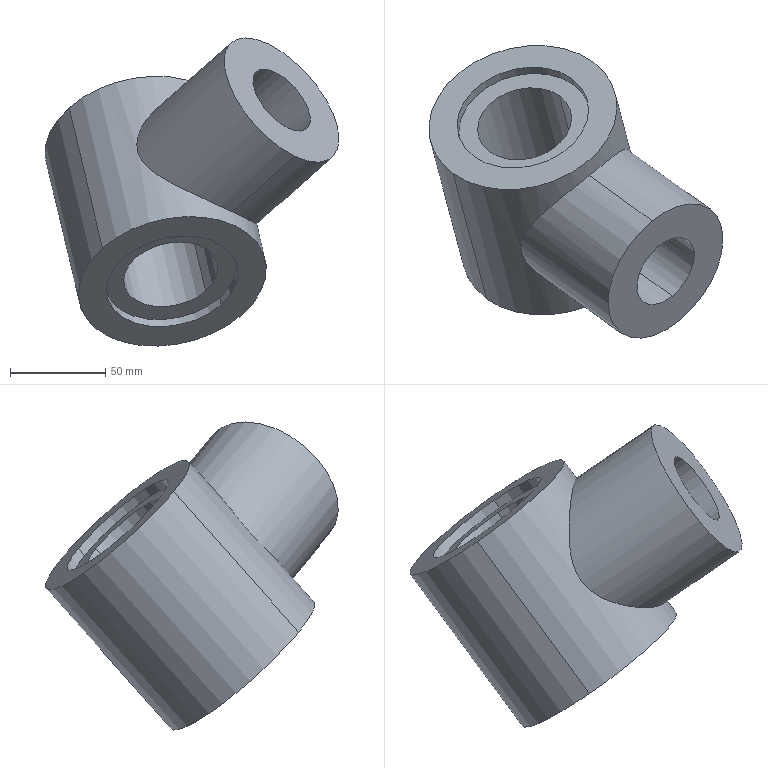Component | SolidWorks | Connector-1 | 1 solid | 18 faces | box 153.98 x 153.34 x 161.37 mm | volume 779589 mm3 | cylinder 13 | plane 5 | commonest cylinder face diameters 70 x4 100 x3 40 x2 80 x2 50 x2 | material Ti-3Al-8V-6Cr-4Mo-4Zr (SS)
build123d program:
from build123d import *

# Parameters (mm, degrees)
SKETCH1_R           = 40
BOSS_EXTRUDE1_DEPTH = 75
SKETCH1_3_R         = 20
CUT_EXTRUDE1_DEPTH  = 65
SKETCH2_R           = 50
BOSS_EXTRUDE2_DEPTH = 50
SKETCH3_R           = 25
CUT_EXTRUDE2_DEPTH  = 50
SKETCH4_R           = 35
CUT_EXTRUDE3_DEPTH  = 5
CUT_EXTRUDE4_START  = -5
SKETCH5_R           = 35
CUT_EXTRUDE4_DEPTH  = 5


with BuildPart() as part:
    # Sketch1 → Boss-Extrude1 (new body)
    with BuildSketch(Plane(origin=(0, 0, 0), x_dir=(1, 0, 0), z_dir=(0, 1, 0))):
        with Locations(Location((0, 0, 0), (0, 0, 270))):
            Circle(SKETCH1_R)
    extrude(amount=BOSS_EXTRUDE1_DEPTH)

    # Sketch1_3 → Cut-Extrude1 (cut)
    with BuildSketch(Plane(origin=(0, 0, 0), x_dir=(1, 0, 0), z_dir=(0, 1, 0))):
        with Locations(Location((0, 0, 0), (0, 0, 270))):
            Circle(SKETCH1_3_R)
    extrude(amount=CUT_EXTRUDE1_DEPTH, mode=Mode.SUBTRACT)

    # Sketch2 → Boss-Extrude2 (add, symmetric)
    with BuildSketch(Plane.XY):
        with Locations((0, 100)):
            Circle(SKETCH2_R)
    extrude(amount=BOSS_EXTRUDE2_DEPTH, both=True)

    # Sketch3 → Cut-Extrude2 (cut, symmetric)
    with BuildSketch(Plane.XY):
        with Locations((0, 100)):
            Circle(SKETCH3_R)
    extrude(amount=CUT_EXTRUDE2_DEPTH, both=True, mode=Mode.SUBTRACT)

    # Sketch4 → Cut-Extrude3 (cut)
    with BuildSketch(Plane(origin=(0, 0, -50), x_dir=(-1, 0, 0), z_dir=(0, 0, -1))):
        with Locations((0, 100)):
            Circle(SKETCH4_R)
    extrude(amount=-CUT_EXTRUDE3_DEPTH, mode=Mode.SUBTRACT)

    # Sketch5 → Cut-Extrude4 (cut)
    with BuildSketch(Plane.XY.offset(50).offset(CUT_EXTRUDE4_START)):
        with Locations(Location((0, 100, 0), (0, 0, 180))):
            Circle(SKETCH5_R)
    extrude(amount=CUT_EXTRUDE4_DEPTH, mode=Mode.SUBTRACT)


solid = part.part

# Placed as in the assembly
solid = solid.moved(Location((-297.638, -1560.033, 10.597), (138.278, 10.084, 137.966)))
STEP:
#1=CARTESIAN_POINT('',(-12.996,-59.896,-3.656));
#2=VERTEX_POINT('',#1);
#3=CARTESIAN_POINT('',(-15.011,-61.512,-2.695));
#4=VERTEX_POINT('',#3);
#5=CARTESIAN_POINT('',(-14.003,-60.704,-3.175));
#6=DIRECTION('',(0.175,-0.6553,-0.7348));
#7=DIRECTION('',(-0.7313,-0.5862,0.3486));
#8=AXIS2_PLACEMENT_3D('',#5,#6,#7);
#9=CIRCLE('',#8,1.378);
#10=EDGE_CURVE('',#2,#4,#9,.T.);
#11=ORIENTED_EDGE('',*,*,#10,.F.);
#12=CARTESIAN_POINT('',(-12.961,-60.025,-3.8));
#13=VERTEX_POINT('',#12);
#14=CARTESIAN_POINT('',(-12.996,-59.896,-3.656));
#15=DIRECTION('',(0.175,-0.6553,-0.7348));
#16=VECTOR('',#15,39.37);
#17=LINE('',#14,#16);
#18=EDGE_CURVE('',#2,#13,#17,.T.);
#19=ORIENTED_EDGE('',*,*,#18,.T.);
#20=CARTESIAN_POINT('',(-14.977,-61.641,-2.84));
#21=VERTEX_POINT('',#20);
#22=CARTESIAN_POINT('',(-13.969,-60.833,-3.32));
#23=DIRECTION('',(0.175,-0.6553,-0.7348));
#24=DIRECTION('',(-0.7313,-0.5862,0.3486));
#25=AXIS2_PLACEMENT_3D('',#22,#23,#24);
#26=CIRCLE('',#25,1.378);
#27=EDGE_CURVE('',#13,#21,#26,.T.);
#28=ORIENTED_EDGE('',*,*,#27,.T.);
#29=CARTESIAN_POINT('',(-15.011,-61.512,-2.695));
#30=DIRECTION('',(0.175,-0.6553,-0.7348));
#31=VECTOR('',#30,39.37);
#32=LINE('',#29,#31);
#33=EDGE_CURVE('',#4,#21,#32,.T.);
#34=ORIENTED_EDGE('',*,*,#33,.F.);
#35=EDGE_LOOP('',(#11,#19,#28,#34));
#36=FACE_OUTER_BOUND('',#35,.T.);
#37=CARTESIAN_POINT('',(-14.003,-60.704,-3.175));
#38=DIRECTION('',(0.175,-0.6553,-0.7348));
#39=DIRECTION('',(-0.7313,-0.5862,0.3486));
#40=AXIS2_PLACEMENT_3D('',#37,#38,#39);
#41=CYLINDRICAL_SURFACE('',#40,1.378);
#42=ADVANCED_FACE('',(#36),#41,.F.);
#43=CARTESIAN_POINT('',(-15.631,-59.19,-0.09136));
#44=VERTEX_POINT('',#43);
#45=CARTESIAN_POINT('',(-13.616,-57.574,-1.052));
#46=VERTEX_POINT('',#45);
#47=CARTESIAN_POINT('',(-14.624,-58.382,-0.5717));
#48=DIRECTION('',(-0.175,0.6553,0.7348));
#49=DIRECTION('',(0.7313,0.5862,-0.3486));
#50=AXIS2_PLACEMENT_3D('',#47,#48,#49);
#51=CIRCLE('',#50,1.378);
#52=EDGE_CURVE('',#44,#46,#51,.T.);
#53=ORIENTED_EDGE('',*,*,#52,.F.);
#54=CARTESIAN_POINT('',(-15.666,-59.061,0.05329));
#55=VERTEX_POINT('',#54);
#56=CARTESIAN_POINT('',(-15.631,-59.19,-0.09136));
#57=DIRECTION('',(-0.175,0.6553,0.7348));
#58=VECTOR('',#57,39.37);
#59=LINE('',#56,#58);
#60=EDGE_CURVE('',#44,#55,#59,.T.);
#61=ORIENTED_EDGE('',*,*,#60,.T.);
#62=CARTESIAN_POINT('',(-13.65,-57.445,-0.9075));
#63=VERTEX_POINT('',#62);
#64=CARTESIAN_POINT('',(-14.658,-58.253,-0.4271));
#65=DIRECTION('',(-0.175,0.6553,0.7348));
#66=DIRECTION('',(0.7313,0.5862,-0.3486));
#67=AXIS2_PLACEMENT_3D('',#64,#65,#66);
#68=CIRCLE('',#67,1.378);
#69=EDGE_CURVE('',#55,#63,#68,.T.);
#70=ORIENTED_EDGE('',*,*,#69,.T.);
#71=CARTESIAN_POINT('',(-13.616,-57.574,-1.052));
#72=DIRECTION('',(-0.175,0.6553,0.7348));
#73=VECTOR('',#72,39.37);
#74=LINE('',#71,#73);
#75=EDGE_CURVE('',#46,#63,#74,.T.);
#76=ORIENTED_EDGE('',*,*,#75,.F.);
#77=EDGE_LOOP('',(#53,#61,#70,#76));
#78=FACE_OUTER_BOUND('',#77,.T.);
#79=CARTESIAN_POINT('',(-14.624,-58.382,-0.5717));
#80=DIRECTION('',(-0.175,0.6553,0.7348));
#81=DIRECTION('',(0.7313,0.5862,-0.3486));
#82=AXIS2_PLACEMENT_3D('',#79,#80,#81);
#83=CYLINDRICAL_SURFACE('',#82,1.378);
#84=ADVANCED_FACE('',(#78),#83,.F.);
#85=CARTESIAN_POINT('',(-13.154,-59.965,-0.1496));
#86=VERTEX_POINT('',#85);
#87=CARTESIAN_POINT('',(-12.878,-60.997,-1.307));
#88=VERTEX_POINT('',#87);
#89=CARTESIAN_POINT('',(-13.154,-59.965,-0.1496));
#90=CARTESIAN_POINT('',(-13.115,-59.934,-0.168));
#91=CARTESIAN_POINT('',(-13.078,-59.906,-0.191));
#92=CARTESIAN_POINT('',(-13.023,-59.869,-0.2323));
#93=CARTESIAN_POINT('',(-13.006,-59.857,-0.2471));
#94=CARTESIAN_POINT('',(-12.979,-59.84,-0.2711));
#95=CARTESIAN_POINT('',(-12.97,-59.835,-0.2794));
#96=CARTESIAN_POINT('',(-12.953,-59.825,-0.2963));
#97=CARTESIAN_POINT('',(-12.945,-59.82,-0.305));
#98=CARTESIAN_POINT('',(-12.903,-59.797,-0.3494));
#99=CARTESIAN_POINT('',(-12.872,-59.782,-0.388));
#100=CARTESIAN_POINT('',(-12.827,-59.766,-0.4503));
#101=CARTESIAN_POINT('',(-12.813,-59.762,-0.4719));
#102=CARTESIAN_POINT('',(-12.785,-59.755,-0.5156));
#103=CARTESIAN_POINT('',(-12.772,-59.753,-0.5379));
#104=CARTESIAN_POINT('',(-12.746,-59.75,-0.5829));
#105=CARTESIAN_POINT('',(-12.734,-59.75,-0.6058));
#106=CARTESIAN_POINT('',(-12.71,-59.752,-0.6521));
#107=CARTESIAN_POINT('',(-12.699,-59.754,-0.6757));
#108=CARTESIAN_POINT('',(-12.666,-59.763,-0.7466));
#109=CARTESIAN_POINT('',(-12.647,-59.774,-0.7935));
#110=CARTESIAN_POINT('',(-12.62,-59.798,-0.8627));
#111=CARTESIAN_POINT('',(-12.612,-59.807,-0.8856));
#112=CARTESIAN_POINT('',(-12.596,-59.827,-0.931));
#113=CARTESIAN_POINT('',(-12.589,-59.839,-0.9535));
#114=CARTESIAN_POINT('',(-12.569,-59.877,-1.019));
#115=CARTESIAN_POINT('',(-12.557,-59.907,-1.06));
#116=CARTESIAN_POINT('',(-12.546,-59.949,-1.108));
#117=CARTESIAN_POINT('',(-12.544,-59.958,-1.117));
#118=CARTESIAN_POINT('',(-12.54,-59.976,-1.135));
#119=CARTESIAN_POINT('',(-12.538,-59.985,-1.144));
#120=CARTESIAN_POINT('',(-12.533,-60.014,-1.171));
#121=CARTESIAN_POINT('',(-12.53,-60.034,-1.187));
#122=CARTESIAN_POINT('',(-12.524,-60.096,-1.234));
#123=CARTESIAN_POINT('',(-12.522,-60.14,-1.262));
#124=CARTESIAN_POINT('',(-12.524,-60.234,-1.309));
#125=CARTESIAN_POINT('',(-12.528,-60.282,-1.328));
#126=CARTESIAN_POINT('',(-12.538,-60.356,-1.351));
#127=CARTESIAN_POINT('',(-12.542,-60.381,-1.358));
#128=CARTESIAN_POINT('',(-12.552,-60.431,-1.37));
#129=CARTESIAN_POINT('',(-12.558,-60.456,-1.374));
#130=CARTESIAN_POINT('',(-12.577,-60.531,-1.386));
#131=CARTESIAN_POINT('',(-12.593,-60.58,-1.39));
#132=CARTESIAN_POINT('',(-12.623,-60.653,-1.391));
#133=CARTESIAN_POINT('',(-12.634,-60.677,-1.39));
#134=CARTESIAN_POINT('',(-12.657,-60.723,-1.387));
#135=CARTESIAN_POINT('',(-12.669,-60.746,-1.385));
#136=CARTESIAN_POINT('',(-12.709,-60.813,-1.375));
#137=CARTESIAN_POINT('',(-12.738,-60.854,-1.366));
#138=CARTESIAN_POINT('',(-12.78,-60.903,-1.35));
#139=CARTESIAN_POINT('',(-12.788,-60.912,-1.347));
#140=CARTESIAN_POINT('',(-12.805,-60.93,-1.339));
#141=CARTESIAN_POINT('',(-12.814,-60.939,-1.336));
#142=CARTESIAN_POINT('',(-12.841,-60.965,-1.324));
#143=CARTESIAN_POINT('',(-12.859,-60.982,-1.316));
#144=CARTESIAN_POINT('',(-12.878,-60.997,-1.307));
#145=B_SPLINE_CURVE_WITH_KNOTS('',3,(#89,#90,#91,#92,#93,#94,#95,#96,#97,#98,#99,#100,#101,#102,#103,#104,#105,#106,#107,#108,#109,#110,#111,#112,#113,#114,#115,#116,#117,#118,#119,#120,#121,#122,#123,#124,#125,#126,#127,#128,#129,#130,#131,#132,#133,#134,#135,#136,#137,#138,#139,#140,#141,#142,#143,#144),.UNSPECIFIED.,.F.,.F.,(4,2,2,2,2,2,2,2,2,2,2,2,2,2,2,2,2,2,2,2,2,2,2,2,2,2,2,4),(0.,0.00395,0.005925,0.006912,0.0079,0.01185,0.01382,0.0158,0.01777,0.01975,0.0237,0.02567,0.02765,0.0316,0.03259,0.03357,0.03555,0.0395,0.04345,0.04542,0.0474,0.05135,0.05332,0.0553,0.05925,0.06024,0.06122,0.0632),.UNSPECIFIED.);
#146=EDGE_CURVE('',#86,#88,#145,.T.);
#147=ORIENTED_EDGE('',*,*,#146,.T.);
#148=CARTESIAN_POINT('',(-11.58,-61.935,-0.1614));
#149=VERTEX_POINT('',#148);
#150=CARTESIAN_POINT('',(-13.267,-60.716,-1.65));
#151=DIRECTION('',(0.6592,-0.4763,0.5818));
#152=VECTOR('',#151,39.37);
#153=LINE('',#150,#152);
#154=EDGE_CURVE('',#88,#149,#153,.T.);
#155=ORIENTED_EDGE('',*,*,#154,.T.);
#156=CARTESIAN_POINT('',(-11.856,-60.903,0.9957));
#157=VERTEX_POINT('',#156);
#158=CARTESIAN_POINT('',(-11.718,-61.419,0.4171));
#159=DIRECTION('',(-0.6592,0.4763,-0.5818));
#160=DIRECTION('',(0.175,-0.6553,-0.7348));
#161=AXIS2_PLACEMENT_3D('',#158,#159,#160);
#162=CIRCLE('',#161,0.7874);
#163=EDGE_CURVE('',#157,#149,#162,.T.);
#164=ORIENTED_EDGE('',*,*,#163,.F.);
#165=CARTESIAN_POINT('',(-13.543,-59.684,-0.4932));
#166=DIRECTION('',(0.6592,-0.4763,0.5818));
#167=VECTOR('',#166,39.37);
#168=LINE('',#165,#167);
#169=EDGE_CURVE('',#86,#157,#168,.T.);
#170=ORIENTED_EDGE('',*,*,#169,.F.);
#171=EDGE_LOOP('',(#147,#155,#164,#170));
#172=FACE_OUTER_BOUND('',#171,.T.);
#173=CARTESIAN_POINT('',(-13.405,-60.2,-1.072));
#174=DIRECTION('',(0.6592,-0.4763,0.5818));
#175=DIRECTION('',(-0.175,0.6553,0.7348));
#176=AXIS2_PLACEMENT_3D('',#173,#174,#175);
#177=CYLINDRICAL_SURFACE('',#176,0.7874);
#178=ADVANCED_FACE('',(#172),#177,.F.);
#179=CARTESIAN_POINT('',(-12.74,-61.513,-1.885));
#180=VERTEX_POINT('',#179);
#181=CARTESIAN_POINT('',(-13.291,-59.449,0.429));
#182=VERTEX_POINT('',#181);
#183=CARTESIAN_POINT('',(-12.74,-61.513,-1.885));
#184=CARTESIAN_POINT('',(-12.78,-61.545,-1.866));
#185=CARTESIAN_POINT('',(-12.821,-61.574,-1.847));
#186=CARTESIAN_POINT('',(-12.887,-61.613,-1.816));
#187=CARTESIAN_POINT('',(-12.91,-61.625,-1.806));
#188=CARTESIAN_POINT('',(-12.955,-61.648,-1.785));
#189=CARTESIAN_POINT('',(-12.978,-61.658,-1.774));
#190=CARTESIAN_POINT('',(-13.047,-61.687,-1.742));
#191=CARTESIAN_POINT('',(-13.094,-61.703,-1.72));
#192=CARTESIAN_POINT('',(-13.166,-61.723,-1.687));
#193=CARTESIAN_POINT('',(-13.19,-61.729,-1.676));
#194=CARTESIAN_POINT('',(-13.24,-61.739,-1.653));
#195=CARTESIAN_POINT('',(-13.264,-61.743,-1.642));
#196=CARTESIAN_POINT('',(-13.388,-61.76,-1.585));
#197=CARTESIAN_POINT('',(-13.487,-61.761,-1.54));
#198=CARTESIAN_POINT('',(-13.61,-61.75,-1.482));
#199=CARTESIAN_POINT('',(-13.635,-61.747,-1.47));
#200=CARTESIAN_POINT('',(-13.684,-61.74,-1.447));
#201=CARTESIAN_POINT('',(-13.708,-61.736,-1.435));
#202=CARTESIAN_POINT('',(-13.781,-61.721,-1.4));
#203=CARTESIAN_POINT('',(-13.829,-61.709,-1.376));
#204=CARTESIAN_POINT('',(-13.922,-61.681,-1.329));
#205=CARTESIAN_POINT('',(-13.969,-61.665,-1.305));
#206=CARTESIAN_POINT('',(-14.036,-61.637,-1.268));
#207=CARTESIAN_POINT('',(-14.059,-61.628,-1.256));
#208=CARTESIAN_POINT('',(-14.103,-61.607,-1.231));
#209=CARTESIAN_POINT('',(-14.125,-61.597,-1.219));
#210=CARTESIAN_POINT('',(-14.19,-61.563,-1.181));
#211=CARTESIAN_POINT('',(-14.231,-61.539,-1.155));
#212=CARTESIAN_POINT('',(-14.311,-61.488,-1.102));
#213=CARTESIAN_POINT('',(-14.349,-61.461,-1.075));
#214=CARTESIAN_POINT('',(-14.422,-61.404,-1.019));
#215=CARTESIAN_POINT('',(-14.456,-61.374,-0.9901));
#216=CARTESIAN_POINT('',(-14.504,-61.326,-0.9439));
#217=CARTESIAN_POINT('',(-14.52,-61.31,-0.9281));
#218=CARTESIAN_POINT('',(-14.549,-61.276,-0.8955));
#219=CARTESIAN_POINT('',(-14.563,-61.26,-0.8788));
#220=CARTESIAN_POINT('',(-14.602,-61.208,-0.8279));
#221=CARTESIAN_POINT('',(-14.625,-61.173,-0.7925));
#222=CARTESIAN_POINT('',(-14.653,-61.12,-0.7366));
#223=CARTESIAN_POINT('',(-14.661,-61.102,-0.7176));
#224=CARTESIAN_POINT('',(-14.672,-61.075,-0.6882));
#225=CARTESIAN_POINT('',(-14.675,-61.066,-0.6783));
#226=CARTESIAN_POINT('',(-14.681,-61.048,-0.6583));
#227=CARTESIAN_POINT('',(-14.684,-61.039,-0.6483));
#228=CARTESIAN_POINT('',(-14.696,-60.994,-0.5979));
#229=CARTESIAN_POINT('',(-14.701,-60.958,-0.5568));
#230=CARTESIAN_POINT('',(-14.702,-60.906,-0.494));
#231=CARTESIAN_POINT('',(-14.701,-60.888,-0.4729));
#232=CARTESIAN_POINT('',(-14.697,-60.854,-0.4304));
#233=CARTESIAN_POINT('',(-14.694,-60.836,-0.409));
#234=CARTESIAN_POINT('',(-14.682,-60.785,-0.3453));
#235=CARTESIAN_POINT('',(-14.671,-60.752,-0.3034));
#236=CARTESIAN_POINT('',(-14.641,-60.687,-0.2209));
#237=CARTESIAN_POINT('',(-14.624,-60.656,-0.1804));
#238=CARTESIAN_POINT('',(-14.593,-60.608,-0.1209));
#239=CARTESIAN_POINT('',(-14.582,-60.592,-0.1012));
#240=CARTESIAN_POINT('',(-14.559,-60.56,-0.06242));
#241=CARTESIAN_POINT('',(-14.547,-60.545,-0.04341));
#242=CARTESIAN_POINT('',(-14.509,-60.498,0.01251));
#243=CARTESIAN_POINT('',(-14.483,-60.467,0.04832));
#244=CARTESIAN_POINT('',(-14.397,-60.374,0.1512));
#245=CARTESIAN_POINT('',(-14.333,-60.313,0.2137));
#246=CARTESIAN_POINT('',(-14.245,-60.233,0.2831));
#247=CARTESIAN_POINT('',(-14.228,-60.217,0.2966));
#248=CARTESIAN_POINT('',(-14.191,-60.185,0.3224));
#249=CARTESIAN_POINT('',(-14.173,-60.169,0.3348));
#250=CARTESIAN_POINT('',(-14.117,-60.12,0.37));
#251=CARTESIAN_POINT('',(-14.079,-60.088,0.3912));
#252=CARTESIAN_POINT('',(-13.963,-59.99,0.4476));
#253=CARTESIAN_POINT('',(-13.882,-59.923,0.4755));
#254=CARTESIAN_POINT('',(-13.776,-59.838,0.4958));
#255=CARTESIAN_POINT('',(-13.755,-59.821,0.4991));
#256=CARTESIAN_POINT('',(-13.712,-59.786,0.5041));
#257=CARTESIAN_POINT('',(-13.691,-59.769,0.5058));
#258=CARTESIAN_POINT('',(-13.627,-59.718,0.5083));
#259=CARTESIAN_POINT('',(-13.585,-59.684,0.5068));
#260=CARTESIAN_POINT('',(-13.5,-59.616,0.4968));
#261=CARTESIAN_POINT('',(-13.457,-59.582,0.4883));
#262=CARTESIAN_POINT('',(-13.394,-59.531,0.47));
#263=CARTESIAN_POINT('',(-13.373,-59.515,0.4631));
#264=CARTESIAN_POINT('',(-13.342,-59.49,0.4513));
#265=CARTESIAN_POINT('',(-13.332,-59.482,0.4471));
#266=CARTESIAN_POINT('',(-13.312,-59.465,0.4384));
#267=CARTESIAN_POINT('',(-13.301,-59.457,0.4338));
#268=CARTESIAN_POINT('',(-13.291,-59.449,0.429));
#269=B_SPLINE_CURVE_WITH_KNOTS('',3,(#183,#184,#185,#186,#187,#188,#189,#190,#191,#192,#193,#194,#195,#196,#197,#198,#199,#200,#201,#202,#203,#204,#205,#206,#207,#208,#209,#210,#211,#212,#213,#214,#215,#216,#217,#218,#219,#220,#221,#222,#223,#224,#225,#226,#227,#228,#229,#230,#231,#232,#233,#234,#235,#236,#237,#238,#239,#240,#241,#242,#243,#244,#245,#246,#247,#248,#249,#250,#251,#252,#253,#254,#255,#256,#257,#258,#259,#260,#261,#262,#263,#264,#265,#266,#267,#268),.UNSPECIFIED.,.F.,.F.,(4,2,2,2,2,2,2,2,2,2,2,2,2,2,2,2,2,2,2,2,2,2,2,2,2,2,2,2,2,2,2,2,2,2,2,2,2,2,2,2,2,2,4),(0.1325,0.1366,0.1386,0.1407,0.1448,0.1469,0.149,0.1572,0.1593,0.1613,0.1655,0.1696,0.1717,0.1737,0.1778,0.182,0.1861,0.1882,0.1902,0.1943,0.1964,0.1974,0.1985,0.2026,0.2047,0.2067,0.2108,0.215,0.217,0.2191,0.2232,0.2315,0.2335,0.2356,0.2397,0.248,0.25,0.2521,0.2562,0.2604,0.2624,0.2635,0.2645),.UNSPECIFIED.);
#270=EDGE_CURVE('',#180,#182,#269,.T.);
#271=ORIENTED_EDGE('',*,*,#270,.F.);
#272=CARTESIAN_POINT('',(-11.442,-62.45,-0.74));
#273=VERTEX_POINT('',#272);
#274=CARTESIAN_POINT('',(-13.389,-61.044,-2.458));
#275=DIRECTION('',(0.6592,-0.4763,0.5818));
#276=VECTOR('',#275,39.37);
#277=LINE('',#274,#276);
#278=EDGE_CURVE('',#180,#273,#277,.T.);
#279=ORIENTED_EDGE('',*,*,#278,.T.);
#280=CARTESIAN_POINT('',(-11.994,-60.387,1.574));
#281=VERTEX_POINT('',#280);
#282=CARTESIAN_POINT('',(-11.718,-61.419,0.4171));
#283=DIRECTION('',(-0.6592,0.4763,-0.5818));
#284=DIRECTION('',(0.175,-0.6553,-0.7348));
#285=AXIS2_PLACEMENT_3D('',#282,#283,#284);
#286=CIRCLE('',#285,1.575);
#287=EDGE_CURVE('',#273,#281,#286,.T.);
#288=ORIENTED_EDGE('',*,*,#287,.T.);
#289=CARTESIAN_POINT('',(-13.94,-58.98,-0.1437));
#290=DIRECTION('',(0.6592,-0.4763,0.5818));
#291=VECTOR('',#290,39.37);
#292=LINE('',#289,#291);
#293=EDGE_CURVE('',#182,#281,#292,.T.);
#294=ORIENTED_EDGE('',*,*,#293,.F.);
#295=EDGE_LOOP('',(#271,#279,#288,#294));
#296=FACE_OUTER_BOUND('',#295,.T.);
#297=CARTESIAN_POINT('',(-13.665,-60.012,-1.301));
#298=DIRECTION('',(0.6592,-0.4763,0.5818));
#299=DIRECTION('',(-0.175,0.6553,0.7348));
#300=AXIS2_PLACEMENT_3D('',#297,#298,#299);
#301=CYLINDRICAL_SURFACE('',#300,1.575);
#302=ADVANCED_FACE('',(#296),#301,.T.);
#303=CARTESIAN_POINT('',(-15.408,-61.987,-2.634));
#304=VERTEX_POINT('',#303);
#305=CARTESIAN_POINT('',(-12.529,-59.679,-4.006));
#306=VERTEX_POINT('',#305);
#307=CARTESIAN_POINT('',(-13.969,-60.833,-3.32));
#308=DIRECTION('',(0.175,-0.6553,-0.7348));
#309=DIRECTION('',(-0.7313,-0.5862,0.3486));
#310=AXIS2_PLACEMENT_3D('',#307,#308,#309);
#311=CIRCLE('',#310,1.969);
#312=EDGE_CURVE('',#304,#306,#311,.T.);
#313=ORIENTED_EDGE('',*,*,#312,.F.);
#314=CARTESIAN_POINT('',(-16.098,-59.407,0.2592));
#315=VERTEX_POINT('',#314);
#316=CARTESIAN_POINT('',(-15.408,-61.987,-2.634));
#317=DIRECTION('',(-0.175,0.6553,0.7348));
#318=VECTOR('',#317,39.37);
#319=LINE('',#316,#318);
#320=EDGE_CURVE('',#304,#315,#319,.T.);
#321=ORIENTED_EDGE('',*,*,#320,.T.);
#322=CARTESIAN_POINT('',(-13.218,-57.099,-1.113));
#323=VERTEX_POINT('',#322);
#324=CARTESIAN_POINT('',(-14.658,-58.253,-0.4271));
#325=DIRECTION('',(0.175,-0.6553,-0.7348));
#326=DIRECTION('',(-0.7313,-0.5862,0.3486));
#327=AXIS2_PLACEMENT_3D('',#324,#325,#326);
#328=CIRCLE('',#327,1.969);
#329=EDGE_CURVE('',#315,#323,#328,.T.);
#330=ORIENTED_EDGE('',*,*,#329,.T.);
#331=CARTESIAN_POINT('',(-12.529,-59.679,-4.006));
#332=DIRECTION('',(-0.175,0.6553,0.7348));
#333=VECTOR('',#332,39.37);
#334=LINE('',#331,#333);
#335=EDGE_CURVE('',#306,#323,#334,.T.);
#336=ORIENTED_EDGE('',*,*,#335,.F.);
#337=EDGE_LOOP('',(#313,#321,#330,#336));
#338=FACE_OUTER_BOUND('',#337,.T.);
#339=CARTESIAN_POINT('',(-13.969,-60.833,-3.32));
#340=DIRECTION('',(-0.175,0.6553,0.7348));
#341=DIRECTION('',(0.7313,0.5862,-0.3486));
#342=AXIS2_PLACEMENT_3D('',#339,#340,#341);
#343=CYLINDRICAL_SURFACE('',#342,1.969);
#344=ADVANCED_FACE('',(#338),#343,.T.);
#345=CARTESIAN_POINT('',(-13.904,-57.805,-0.9149));
#346=VERTEX_POINT('',#345);
#347=CARTESIAN_POINT('',(-15.343,-58.959,-0.2286));
#348=VERTEX_POINT('',#347);
#349=CARTESIAN_POINT('',(-14.624,-58.382,-0.5717));
#350=DIRECTION('',(0.175,-0.6553,-0.7348));
#351=DIRECTION('',(0.7313,0.5862,-0.3486));
#352=AXIS2_PLACEMENT_3D('',#349,#350,#351);
#353=CIRCLE('',#352,0.9843);
#354=EDGE_CURVE('',#346,#348,#353,.T.);
#355=ORIENTED_EDGE('',*,*,#354,.F.);
#356=CARTESIAN_POINT('',(-13.284,-60.127,-3.518));
#357=VERTEX_POINT('',#356);
#358=CARTESIAN_POINT('',(-13.938,-57.676,-0.7702));
#359=DIRECTION('',(0.175,-0.6553,-0.7348));
#360=VECTOR('',#359,39.37);
#361=LINE('',#358,#360);
#362=EDGE_CURVE('',#346,#357,#361,.T.);
#363=ORIENTED_EDGE('',*,*,#362,.T.);
#364=CARTESIAN_POINT('',(-14.723,-61.281,-2.832));
#365=VERTEX_POINT('',#364);
#366=CARTESIAN_POINT('',(-14.003,-60.704,-3.175));
#367=DIRECTION('',(-0.175,0.6553,0.7348));
#368=DIRECTION('',(-0.7313,-0.5862,0.3486));
#369=AXIS2_PLACEMENT_3D('',#366,#367,#368);
#370=CIRCLE('',#369,0.9843);
#371=EDGE_CURVE('',#365,#357,#370,.T.);
#372=ORIENTED_EDGE('',*,*,#371,.F.);
#373=CARTESIAN_POINT('',(-15.378,-58.83,-0.08396));
#374=DIRECTION('',(0.175,-0.6553,-0.7348));
#375=VECTOR('',#374,39.37);
#376=LINE('',#373,#375);
#377=EDGE_CURVE('',#348,#365,#376,.T.);
#378=ORIENTED_EDGE('',*,*,#377,.F.);
#379=EDGE_LOOP('',(#355,#363,#372,#378));
#380=FACE_OUTER_BOUND('',#379,.T.);
#381=CARTESIAN_POINT('',(-14.658,-58.253,-0.4271));
#382=DIRECTION('',(0.175,-0.6553,-0.7348));
#383=DIRECTION('',(-0.7313,-0.5862,0.3486));
#384=AXIS2_PLACEMENT_3D('',#381,#382,#383);
#385=CYLINDRICAL_SURFACE('',#384,0.9843);
#386=ADVANCED_FACE('',(#380),#385,.F.);
#387=ORIENTED_EDGE('',*,*,#362,.F.);
#388=CARTESIAN_POINT('',(-14.624,-58.382,-0.5717));
#389=DIRECTION('',(0.175,-0.6553,-0.7348));
#390=DIRECTION('',(0.7313,0.5862,-0.3486));
#391=AXIS2_PLACEMENT_3D('',#388,#389,#390);
#392=CIRCLE('',#391,0.9843);
#393=EDGE_CURVE('',#348,#346,#392,.T.);
#394=ORIENTED_EDGE('',*,*,#393,.F.);
#395=ORIENTED_EDGE('',*,*,#377,.T.);
#396=CARTESIAN_POINT('',(-14.003,-60.704,-3.175));
#397=DIRECTION('',(-0.175,0.6553,0.7348));
#398=DIRECTION('',(-0.7313,-0.5862,0.3486));
#399=AXIS2_PLACEMENT_3D('',#396,#397,#398);
#400=CIRCLE('',#399,0.9843);
#401=EDGE_CURVE('',#357,#365,#400,.T.);
#402=ORIENTED_EDGE('',*,*,#401,.F.);
#403=EDGE_LOOP('',(#387,#394,#395,#402));
#404=FACE_OUTER_BOUND('',#403,.T.);
#405=CARTESIAN_POINT('',(-14.658,-58.253,-0.4271));
#406=DIRECTION('',(0.175,-0.6553,-0.7348));
#407=DIRECTION('',(-0.7313,-0.5862,0.3486));
#408=AXIS2_PLACEMENT_3D('',#405,#406,#407);
#409=CYLINDRICAL_SURFACE('',#408,0.9843);
#410=ADVANCED_FACE('',(#404),#409,.F.);
#411=ORIENTED_EDGE('',*,*,#320,.F.);
#412=CARTESIAN_POINT('',(-13.969,-60.833,-3.32));
#413=DIRECTION('',(0.175,-0.6553,-0.7348));
#414=DIRECTION('',(-0.7313,-0.5862,0.3486));
#415=AXIS2_PLACEMENT_3D('',#412,#413,#414);
#416=CIRCLE('',#415,1.969);
#417=EDGE_CURVE('',#306,#304,#416,.T.);
#418=ORIENTED_EDGE('',*,*,#417,.F.);
#419=ORIENTED_EDGE('',*,*,#335,.T.);
#420=CARTESIAN_POINT('',(-14.658,-58.253,-0.4271));
#421=DIRECTION('',(0.175,-0.6553,-0.7348));
#422=DIRECTION('',(-0.7313,-0.5862,0.3486));
#423=AXIS2_PLACEMENT_3D('',#420,#421,#422);
#424=CIRCLE('',#423,1.969);
#425=EDGE_CURVE('',#323,#315,#424,.T.);
#426=ORIENTED_EDGE('',*,*,#425,.T.);
#427=EDGE_LOOP('',(#411,#418,#419,#426));
#428=FACE_OUTER_BOUND('',#427,.T.);
#429=CARTESIAN_POINT('',(-13.291,-59.449,0.429));
#430=CARTESIAN_POINT('',(-13.211,-59.384,0.3905));
#431=CARTESIAN_POINT('',(-13.136,-59.324,0.3391));
#432=CARTESIAN_POINT('',(-13.049,-59.255,0.2601));
#433=CARTESIAN_POINT('',(-13.032,-59.241,0.2436));
#434=CARTESIAN_POINT('',(-12.999,-59.214,0.2091));
#435=CARTESIAN_POINT('',(-12.983,-59.201,0.191));
#436=CARTESIAN_POINT('',(-12.935,-59.163,0.1353));
#437=CARTESIAN_POINT('',(-12.905,-59.14,0.09602));
#438=CARTESIAN_POINT('',(-12.85,-59.096,0.01354));
#439=CARTESIAN_POINT('',(-12.823,-59.075,-0.02965));
#440=CARTESIAN_POINT('',(-12.774,-59.037,-0.1197));
#441=CARTESIAN_POINT('',(-12.751,-59.02,-0.1668));
#442=CARTESIAN_POINT('',(-12.687,-58.973,-0.3104));
#443=CARTESIAN_POINT('',(-12.651,-58.949,-0.41));
#444=CARTESIAN_POINT('',(-12.604,-58.923,-0.5643));
#445=CARTESIAN_POINT('',(-12.59,-58.916,-0.6165));
#446=CARTESIAN_POINT('',(-12.57,-58.909,-0.6959));
#447=CARTESIAN_POINT('',(-12.564,-58.907,-0.7227));
#448=CARTESIAN_POINT('',(-12.552,-58.904,-0.7761));
#449=CARTESIAN_POINT('',(-12.546,-58.903,-0.8028));
#450=CARTESIAN_POINT('',(-12.53,-58.902,-0.8829));
#451=CARTESIAN_POINT('',(-12.519,-58.903,-0.9362));
#452=CARTESIAN_POINT('',(-12.501,-58.91,-1.043));
#453=CARTESIAN_POINT('',(-12.492,-58.916,-1.096));
#454=CARTESIAN_POINT('',(-12.475,-58.933,-1.202));
#455=CARTESIAN_POINT('',(-12.467,-58.944,-1.255));
#456=CARTESIAN_POINT('',(-12.455,-58.965,-1.334));
#457=CARTESIAN_POINT('',(-12.451,-58.974,-1.36));
#458=CARTESIAN_POINT('',(-12.444,-58.991,-1.411));
#459=CARTESIAN_POINT('',(-12.44,-59.001,-1.437));
#460=CARTESIAN_POINT('',(-12.428,-59.032,-1.511));
#461=CARTESIAN_POINT('',(-12.419,-59.057,-1.559));
#462=CARTESIAN_POINT('',(-12.406,-59.1,-1.629));
#463=CARTESIAN_POINT('',(-12.402,-59.116,-1.651));
#464=CARTESIAN_POINT('',(-12.393,-59.148,-1.695));
#465=CARTESIAN_POINT('',(-12.388,-59.165,-1.716));
#466=CARTESIAN_POINT('',(-12.374,-59.219,-1.776));
#467=CARTESIAN_POINT('',(-12.364,-59.258,-1.812));
#468=CARTESIAN_POINT('',(-12.348,-59.321,-1.862));
#469=CARTESIAN_POINT('',(-12.343,-59.343,-1.878));
#470=CARTESIAN_POINT('',(-12.333,-59.388,-1.908));
#471=CARTESIAN_POINT('',(-12.328,-59.411,-1.923));
#472=CARTESIAN_POINT('',(-12.312,-59.481,-1.962));
#473=CARTESIAN_POINT('',(-12.303,-59.53,-1.985));
#474=CARTESIAN_POINT('',(-12.289,-59.605,-2.015));
#475=CARTESIAN_POINT('',(-12.284,-59.63,-2.024));
#476=CARTESIAN_POINT('',(-12.275,-59.681,-2.041));
#477=CARTESIAN_POINT('',(-12.271,-59.707,-2.049));
#478=CARTESIAN_POINT('',(-12.26,-59.786,-2.072));
#479=CARTESIAN_POINT('',(-12.253,-59.839,-2.084));
#480=CARTESIAN_POINT('',(-12.241,-59.945,-2.104));
#481=CARTESIAN_POINT('',(-12.237,-59.999,-2.112));
#482=CARTESIAN_POINT('',(-12.23,-60.106,-2.124));
#483=CARTESIAN_POINT('',(-12.229,-60.161,-2.129));
#484=CARTESIAN_POINT('',(-12.229,-60.242,-2.133));
#485=CARTESIAN_POINT('',(-12.229,-60.27,-2.134));
#486=CARTESIAN_POINT('',(-12.23,-60.325,-2.135));
#487=CARTESIAN_POINT('',(-12.232,-60.352,-2.136));
#488=CARTESIAN_POINT('',(-12.24,-60.489,-2.135));
#489=CARTESIAN_POINT('',(-12.254,-60.596,-2.129));
#490=CARTESIAN_POINT('',(-12.287,-60.754,-2.112));
#491=CARTESIAN_POINT('',(-12.301,-60.807,-2.105));
#492=CARTESIAN_POINT('',(-12.325,-60.884,-2.093));
#493=CARTESIAN_POINT('',(-12.333,-60.91,-2.088));
#494=CARTESIAN_POINT('',(-12.352,-60.961,-2.079));
#495=CARTESIAN_POINT('',(-12.361,-60.986,-2.073));
#496=CARTESIAN_POINT('',(-12.414,-61.11,-2.046));
#497=CARTESIAN_POINT('',(-12.465,-61.203,-2.02));
#498=CARTESIAN_POINT('',(-12.542,-61.309,-1.982));
#499=CARTESIAN_POINT('',(-12.558,-61.33,-1.974));
#500=CARTESIAN_POINT('',(-12.592,-61.37,-1.957));
#501=CARTESIAN_POINT('',(-12.609,-61.39,-1.949));
#502=CARTESIAN_POINT('',(-12.663,-61.446,-1.922));
#503=CARTESIAN_POINT('',(-12.7,-61.481,-1.904));
#504=CARTESIAN_POINT('',(-12.74,-61.513,-1.885));
#505=B_SPLINE_CURVE_WITH_KNOTS('',3,(#429,#430,#431,#432,#433,#434,#435,#436,#437,#438,#439,#440,#441,#442,#443,#444,#445,#446,#447,#448,#449,#450,#451,#452,#453,#454,#455,#456,#457,#458,#459,#460,#461,#462,#463,#464,#465,#466,#467,#468,#469,#470,#471,#472,#473,#474,#475,#476,#477,#478,#479,#480,#481,#482,#483,#484,#485,#486,#487,#488,#489,#490,#491,#492,#493,#494,#495,#496,#497,#498,#499,#500,#501,#502,#503,#504),.UNSPECIFIED.,.F.,.F.,(4,2,2,2,2,2,2,2,2,2,2,2,2,2,2,2,2,2,2,2,2,2,2,2,2,2,2,2,2,2,2,2,2,2,2,2,2,4),(0.,0.008279,0.01035,0.01242,0.01656,0.0207,0.02484,0.03311,0.03725,0.03932,0.04139,0.04553,0.04967,0.05381,0.05588,0.05795,0.06209,0.06416,0.06623,0.07037,0.07244,0.07451,0.07865,0.08072,0.08279,0.08693,0.09106,0.0952,0.09727,0.09934,0.1076,0.1118,0.1138,0.1159,0.1242,0.1262,0.1283,0.1325),.UNSPECIFIED.);
#506=EDGE_CURVE('',#182,#180,#505,.T.);
#507=ORIENTED_EDGE('',*,*,#506,.T.);
#508=ORIENTED_EDGE('',*,*,#270,.T.);
#509=EDGE_LOOP('',(#507,#508));
#510=FACE_BOUND('',#509,.T.);
#511=CARTESIAN_POINT('',(-13.969,-60.833,-3.32));
#512=DIRECTION('',(-0.175,0.6553,0.7348));
#513=DIRECTION('',(0.7313,0.5862,-0.3486));
#514=AXIS2_PLACEMENT_3D('',#511,#512,#513);
#515=CYLINDRICAL_SURFACE('',#514,1.969);
#516=ADVANCED_FACE('',(#428,#510),#515,.T.);
#517=CARTESIAN_POINT('',(-13.969,-60.833,-3.32));
#518=DIRECTION('',(0.175,-0.6553,-0.7348));
#519=DIRECTION('',(-0.7313,-0.5862,0.3486));
#520=AXIS2_PLACEMENT_3D('',#517,#518,#519);
#521=CIRCLE('',#520,1.378);
#522=EDGE_CURVE('',#21,#13,#521,.T.);
#523=ORIENTED_EDGE('',*,*,#522,.F.);
#524=ORIENTED_EDGE('',*,*,#27,.F.);
#525=EDGE_LOOP('',(#523,#524));
#526=FACE_BOUND('',#525,.T.);
#527=ORIENTED_EDGE('',*,*,#417,.T.);
#528=ORIENTED_EDGE('',*,*,#312,.T.);
#529=EDGE_LOOP('',(#527,#528));
#530=FACE_OUTER_BOUND('',#529,.T.);
#531=CARTESIAN_POINT('',(-13.969,-60.833,-3.32));
#532=DIRECTION('',(0.175,-0.6553,-0.7348));
#533=DIRECTION('',(-0.7313,-0.5862,0.3486));
#534=AXIS2_PLACEMENT_3D('',#531,#532,#533);
#535=PLANE('',#534);
#536=ADVANCED_FACE('',(#526,#530),#535,.T.);
#537=CARTESIAN_POINT('',(-14.658,-58.253,-0.4271));
#538=DIRECTION('',(-0.175,0.6553,0.7348));
#539=DIRECTION('',(0.7313,0.5862,-0.3486));
#540=AXIS2_PLACEMENT_3D('',#537,#538,#539);
#541=CIRCLE('',#540,1.378);
#542=EDGE_CURVE('',#63,#55,#541,.T.);
#543=ORIENTED_EDGE('',*,*,#542,.F.);
#544=ORIENTED_EDGE('',*,*,#69,.F.);
#545=EDGE_LOOP('',(#543,#544));
#546=FACE_BOUND('',#545,.T.);
#547=ORIENTED_EDGE('',*,*,#425,.F.);
#548=ORIENTED_EDGE('',*,*,#329,.F.);
#549=EDGE_LOOP('',(#547,#548));
#550=FACE_OUTER_BOUND('',#549,.T.);
#551=CARTESIAN_POINT('',(-14.658,-58.253,-0.4271));
#552=DIRECTION('',(0.175,-0.6553,-0.7348));
#553=DIRECTION('',(-0.7313,-0.5862,0.3486));
#554=AXIS2_PLACEMENT_3D('',#551,#552,#553);
#555=PLANE('',#554);
#556=ADVANCED_FACE('',(#546,#550),#555,.F.);
#557=ORIENTED_EDGE('',*,*,#278,.F.);
#558=ORIENTED_EDGE('',*,*,#506,.F.);
#559=ORIENTED_EDGE('',*,*,#293,.T.);
#560=CARTESIAN_POINT('',(-11.718,-61.419,0.4171));
#561=DIRECTION('',(-0.6592,0.4763,-0.5818));
#562=DIRECTION('',(0.175,-0.6553,-0.7348));
#563=AXIS2_PLACEMENT_3D('',#560,#561,#562);
#564=CIRCLE('',#563,1.575);
#565=EDGE_CURVE('',#281,#273,#564,.T.);
#566=ORIENTED_EDGE('',*,*,#565,.T.);
#567=EDGE_LOOP('',(#557,#558,#559,#566));
#568=FACE_OUTER_BOUND('',#567,.T.);
#569=CARTESIAN_POINT('',(-13.665,-60.012,-1.301));
#570=DIRECTION('',(0.6592,-0.4763,0.5818));
#571=DIRECTION('',(-0.175,0.6553,0.7348));
#572=AXIS2_PLACEMENT_3D('',#569,#570,#571);
#573=CYLINDRICAL_SURFACE('',#572,1.575);
#574=ADVANCED_FACE('',(#568),#573,.T.);
#575=ORIENTED_EDGE('',*,*,#154,.F.);
#576=CARTESIAN_POINT('',(-12.878,-60.997,-1.307));
#577=CARTESIAN_POINT('',(-12.897,-61.012,-1.298));
#578=CARTESIAN_POINT('',(-12.916,-61.026,-1.288));
#579=CARTESIAN_POINT('',(-12.957,-61.052,-1.267));
#580=CARTESIAN_POINT('',(-12.977,-61.064,-1.256));
#581=CARTESIAN_POINT('',(-13.04,-61.096,-1.222));
#582=CARTESIAN_POINT('',(-13.083,-61.112,-1.197));
#583=CARTESIAN_POINT('',(-13.147,-61.129,-1.157));
#584=CARTESIAN_POINT('',(-13.169,-61.134,-1.143));
#585=CARTESIAN_POINT('',(-13.213,-61.14,-1.114));
#586=CARTESIAN_POINT('',(-13.234,-61.142,-1.099));
#587=CARTESIAN_POINT('',(-13.276,-61.144,-1.069));
#588=CARTESIAN_POINT('',(-13.297,-61.143,-1.054));
#589=CARTESIAN_POINT('',(-13.339,-61.14,-1.022));
#590=CARTESIAN_POINT('',(-13.359,-61.138,-1.006));
#591=CARTESIAN_POINT('',(-13.419,-61.126,-0.9565));
#592=CARTESIAN_POINT('',(-13.456,-61.114,-0.9226));
#593=CARTESIAN_POINT('',(-13.508,-61.09,-0.8699));
#594=CARTESIAN_POINT('',(-13.525,-61.082,-0.852));
#595=CARTESIAN_POINT('',(-13.557,-61.062,-0.8155));
#596=CARTESIAN_POINT('',(-13.572,-61.051,-0.7969));
#597=CARTESIAN_POINT('',(-13.614,-61.016,-0.741));
#598=CARTESIAN_POINT('',(-13.638,-60.99,-0.7034));
#599=CARTESIAN_POINT('',(-13.667,-60.946,-0.646));
#600=CARTESIAN_POINT('',(-13.675,-60.93,-0.6266));
#601=CARTESIAN_POINT('',(-13.69,-60.898,-0.5877));
#602=CARTESIAN_POINT('',(-13.695,-60.881,-0.5685));
#603=CARTESIAN_POINT('',(-13.709,-60.83,-0.5113));
#604=CARTESIAN_POINT('',(-13.713,-60.795,-0.4738));
#605=CARTESIAN_POINT('',(-13.711,-60.748,-0.428));
#606=CARTESIAN_POINT('',(-13.71,-60.738,-0.4189));
#607=CARTESIAN_POINT('',(-13.708,-60.719,-0.401));
#608=CARTESIAN_POINT('',(-13.707,-60.71,-0.3922));
#609=CARTESIAN_POINT('',(-13.702,-60.681,-0.3662));
#610=CARTESIAN_POINT('',(-13.698,-60.662,-0.3494));
#611=CARTESIAN_POINT('',(-13.686,-60.623,-0.3169));
#612=CARTESIAN_POINT('',(-13.679,-60.603,-0.3012));
#613=CARTESIAN_POINT('',(-13.664,-60.563,-0.271));
#614=CARTESIAN_POINT('',(-13.654,-60.543,-0.2565));
#615=CARTESIAN_POINT('',(-13.624,-60.484,-0.2158));
#616=CARTESIAN_POINT('',(-13.601,-60.444,-0.1921));
#617=CARTESIAN_POINT('',(-13.56,-60.384,-0.1618));
#618=CARTESIAN_POINT('',(-13.546,-60.364,-0.1526));
#619=CARTESIAN_POINT('',(-13.515,-60.325,-0.1365));
#620=CARTESIAN_POINT('',(-13.5,-60.305,-0.1295));
#621=CARTESIAN_POINT('',(-13.451,-60.247,-0.1119));
#622=CARTESIAN_POINT('',(-13.417,-60.209,-0.1046));
#623=CARTESIAN_POINT('',(-13.362,-60.153,-0.101));
#624=CARTESIAN_POINT('',(-13.344,-60.134,-0.1011));
#625=CARTESIAN_POINT('',(-13.306,-60.098,-0.1039));
#626=CARTESIAN_POINT('',(-13.287,-60.08,-0.1065));
#627=CARTESIAN_POINT('',(-13.25,-60.046,-0.1143));
#628=CARTESIAN_POINT('',(-13.231,-60.029,-0.1195));
#629=CARTESIAN_POINT('',(-13.192,-59.996,-0.1326));
#630=CARTESIAN_POINT('',(-13.173,-59.98,-0.1405));
#631=CARTESIAN_POINT('',(-13.154,-59.965,-0.1496));
#632=B_SPLINE_CURVE_WITH_KNOTS('',3,(#576,#577,#578,#579,#580,#581,#582,#583,#584,#585,#586,#587,#588,#589,#590,#591,#592,#593,#594,#595,#596,#597,#598,#599,#600,#601,#602,#603,#604,#605,#606,#607,#608,#609,#610,#611,#612,#613,#614,#615,#616,#617,#618,#619,#620,#621,#622,#623,#624,#625,#626,#627,#628,#629,#630,#631),.UNSPECIFIED.,.F.,.F.,(4,2,2,2,2,2,2,2,2,2,2,2,2,2,2,2,2,2,2,2,2,2,2,2,2,2,2,4),(0.0632,0.06517,0.06715,0.07109,0.07307,0.07504,0.07701,0.07899,0.08293,0.08491,0.08688,0.09083,0.0928,0.09478,0.09872,0.09971,0.1007,0.1027,0.1046,0.1066,0.1106,0.1125,0.1145,0.1185,0.1204,0.1224,0.1244,0.1264),.UNSPECIFIED.);
#633=EDGE_CURVE('',#88,#86,#632,.T.);
#634=ORIENTED_EDGE('',*,*,#633,.T.);
#635=ORIENTED_EDGE('',*,*,#169,.T.);
#636=CARTESIAN_POINT('',(-11.718,-61.419,0.4171));
#637=DIRECTION('',(-0.6592,0.4763,-0.5818));
#638=DIRECTION('',(0.175,-0.6553,-0.7348));
#639=AXIS2_PLACEMENT_3D('',#636,#637,#638);
#640=CIRCLE('',#639,0.7874);
#641=EDGE_CURVE('',#149,#157,#640,.T.);
#642=ORIENTED_EDGE('',*,*,#641,.F.);
#643=EDGE_LOOP('',(#575,#634,#635,#642));
#644=FACE_OUTER_BOUND('',#643,.T.);
#645=CARTESIAN_POINT('',(-13.405,-60.2,-1.072));
#646=DIRECTION('',(0.6592,-0.4763,0.5818));
#647=DIRECTION('',(-0.175,0.6553,0.7348));
#648=AXIS2_PLACEMENT_3D('',#645,#646,#647);
#649=CYLINDRICAL_SURFACE('',#648,0.7874);
#650=ADVANCED_FACE('',(#644),#649,.F.);
#651=ORIENTED_EDGE('',*,*,#163,.T.);
#652=ORIENTED_EDGE('',*,*,#641,.T.);
#653=EDGE_LOOP('',(#651,#652));
#654=FACE_BOUND('',#653,.T.);
#655=ORIENTED_EDGE('',*,*,#565,.F.);
#656=ORIENTED_EDGE('',*,*,#287,.F.);
#657=EDGE_LOOP('',(#655,#656));
#658=FACE_OUTER_BOUND('',#657,.T.);
#659=CARTESIAN_POINT('',(-11.718,-61.419,0.4171));
#660=DIRECTION('',(-0.6592,0.4763,-0.5818));
#661=DIRECTION('',(0.175,-0.6553,-0.7348));
#662=AXIS2_PLACEMENT_3D('',#659,#660,#661);
#663=PLANE('',#662);
#664=ADVANCED_FACE('',(#654,#658),#663,.F.);
#665=ORIENTED_EDGE('',*,*,#146,.F.);
#666=ORIENTED_EDGE('',*,*,#633,.F.);
#667=EDGE_LOOP('',(#665,#666));
#668=FACE_OUTER_BOUND('',#667,.T.);
#669=CARTESIAN_POINT('',(-13.969,-60.833,-3.32));
#670=DIRECTION('',(-0.175,0.6553,0.7348));
#671=DIRECTION('',(0.7313,0.5862,-0.3486));
#672=AXIS2_PLACEMENT_3D('',#669,#670,#671);
#673=CYLINDRICAL_SURFACE('',#672,1.969);
#674=ADVANCED_FACE('',(#668),#673,.T.);
#675=CARTESIAN_POINT('',(-14.624,-58.382,-0.5717));
#676=DIRECTION('',(-0.175,0.6553,0.7348));
#677=DIRECTION('',(0.7313,0.5862,-0.3486));
#678=AXIS2_PLACEMENT_3D('',#675,#676,#677);
#679=CIRCLE('',#678,1.378);
#680=EDGE_CURVE('',#46,#44,#679,.T.);
#681=ORIENTED_EDGE('',*,*,#680,.T.);
#682=ORIENTED_EDGE('',*,*,#52,.T.);
#683=EDGE_LOOP('',(#681,#682));
#684=FACE_OUTER_BOUND('',#683,.T.);
#685=ORIENTED_EDGE('',*,*,#393,.T.);
#686=ORIENTED_EDGE('',*,*,#354,.T.);
#687=EDGE_LOOP('',(#685,#686));
#688=FACE_BOUND('',#687,.T.);
#689=CARTESIAN_POINT('',(-14.624,-58.382,-0.5717));
#690=DIRECTION('',(-0.175,0.6553,0.7348));
#691=DIRECTION('',(0.7313,0.5862,-0.3486));
#692=AXIS2_PLACEMENT_3D('',#689,#690,#691);
#693=PLANE('',#692);
#694=ADVANCED_FACE('',(#684,#688),#693,.T.);
#695=ORIENTED_EDGE('',*,*,#60,.F.);
#696=ORIENTED_EDGE('',*,*,#680,.F.);
#697=ORIENTED_EDGE('',*,*,#75,.T.);
#698=ORIENTED_EDGE('',*,*,#542,.T.);
#699=EDGE_LOOP('',(#695,#696,#697,#698));
#700=FACE_OUTER_BOUND('',#699,.T.);
#701=CARTESIAN_POINT('',(-14.624,-58.382,-0.5717));
#702=DIRECTION('',(-0.175,0.6553,0.7348));
#703=DIRECTION('',(0.7313,0.5862,-0.3486));
#704=AXIS2_PLACEMENT_3D('',#701,#702,#703);
#705=CYLINDRICAL_SURFACE('',#704,1.378);
#706=ADVANCED_FACE('',(#700),#705,.F.);
#707=CARTESIAN_POINT('',(-14.003,-60.704,-3.175));
#708=DIRECTION('',(0.175,-0.6553,-0.7348));
#709=DIRECTION('',(-0.7313,-0.5862,0.3486));
#710=AXIS2_PLACEMENT_3D('',#707,#708,#709);
#711=CIRCLE('',#710,1.378);
#712=EDGE_CURVE('',#4,#2,#711,.T.);
#713=ORIENTED_EDGE('',*,*,#712,.T.);
#714=ORIENTED_EDGE('',*,*,#10,.T.);
#715=EDGE_LOOP('',(#713,#714));
#716=FACE_OUTER_BOUND('',#715,.T.);
#717=ORIENTED_EDGE('',*,*,#371,.T.);
#718=ORIENTED_EDGE('',*,*,#401,.T.);
#719=EDGE_LOOP('',(#717,#718));
#720=FACE_BOUND('',#719,.T.);
#721=CARTESIAN_POINT('',(-14.003,-60.704,-3.175));
#722=DIRECTION('',(0.175,-0.6553,-0.7348));
#723=DIRECTION('',(-0.7313,-0.5862,0.3486));
#724=AXIS2_PLACEMENT_3D('',#721,#722,#723);
#725=PLANE('',#724);
#726=ADVANCED_FACE('',(#716,#720),#725,.T.);
#727=ORIENTED_EDGE('',*,*,#18,.F.);
#728=ORIENTED_EDGE('',*,*,#712,.F.);
#729=ORIENTED_EDGE('',*,*,#33,.T.);
#730=ORIENTED_EDGE('',*,*,#522,.T.);
#731=EDGE_LOOP('',(#727,#728,#729,#730));
#732=FACE_OUTER_BOUND('',#731,.T.);
#733=CARTESIAN_POINT('',(-14.003,-60.704,-3.175));
#734=DIRECTION('',(0.175,-0.6553,-0.7348));
#735=DIRECTION('',(-0.7313,-0.5862,0.3486));
#736=AXIS2_PLACEMENT_3D('',#733,#734,#735);
#737=CYLINDRICAL_SURFACE('',#736,1.378);
#738=ADVANCED_FACE('',(#732),#737,.F.);
#739=CLOSED_SHELL('',(#42,#84,#178,#302,#344,#386,#410,#516,#536,#556,#574,#650,#664,#674,#694,#706,#726,#738));
#740=MANIFOLD_SOLID_BREP('',#739);
#741=CARTESIAN_POINT('',(0.,0.,0.));
#742=DIRECTION('',(0.,0.,1.));
#743=DIRECTION('',(1.,0.,0.));
#744=AXIS2_PLACEMENT_3D('',#741,#742,#743);
#745=(LENGTH_UNIT()NAMED_UNIT(*)SI_UNIT($,.METRE.));
#746=LENGTH_MEASURE_WITH_UNIT(LENGTH_MEASURE(0.0254),#745);
#747=DIMENSIONAL_EXPONENTS(1.,0.,0.,0.,0.,0.,0.);
#748=(CONVERSION_BASED_UNIT('',#746)LENGTH_UNIT()NAMED_UNIT(#747));
#749=UNCERTAINTY_MEASURE_WITH_UNIT(LENGTH_MEASURE(0.00001),#748,'','');
#750=(NAMED_UNIT(*)PLANE_ANGLE_UNIT()SI_UNIT($,.RADIAN.));
#751=(NAMED_UNIT(*)SI_UNIT($,.STERADIAN.)SOLID_ANGLE_UNIT());
#752=(GEOMETRIC_REPRESENTATION_CONTEXT(3)GLOBAL_UNCERTAINTY_ASSIGNED_CONTEXT((#749))GLOBAL_UNIT_ASSIGNED_CONTEXT((#748,#750,#751))REPRESENTATION_CONTEXT('',''));
#753=ADVANCED_BREP_SHAPE_REPRESENTATION('',(#740,#744),#752);
#754=COLOUR_RGB('',0.7922,0.8196,0.9333);
#755=FILL_AREA_STYLE_COLOUR('',#754);
#756=FILL_AREA_STYLE('',(#755));
#757=SURFACE_STYLE_FILL_AREA(#756);
#758=SURFACE_SIDE_STYLE('',(#757));
#759=SURFACE_STYLE_USAGE(.BOTH.,#758);
#760=PRESENTATION_STYLE_ASSIGNMENT((#759));
#761=STYLED_ITEM('',(#760),#740);
#762=PRESENTATION_LAYER_ASSIGNMENT('','',(#761));
#763=(LENGTH_UNIT()NAMED_UNIT(*)SI_UNIT($,.METRE.));
#764=LENGTH_MEASURE_WITH_UNIT(LENGTH_MEASURE(0.0254),#763);
#765=DIMENSIONAL_EXPONENTS(1.,0.,0.,0.,0.,0.,0.);
#766=(CONVERSION_BASED_UNIT('',#764)LENGTH_UNIT()NAMED_UNIT(#765));
#767=UNCERTAINTY_MEASURE_WITH_UNIT(LENGTH_MEASURE(0.00001),#766,'','');
#768=(NAMED_UNIT(*)PLANE_ANGLE_UNIT()SI_UNIT($,.RADIAN.));
#769=(NAMED_UNIT(*)SI_UNIT($,.STERADIAN.)SOLID_ANGLE_UNIT());
#770=(GEOMETRIC_REPRESENTATION_CONTEXT(3)GLOBAL_UNCERTAINTY_ASSIGNED_CONTEXT((#767))GLOBAL_UNIT_ASSIGNED_CONTEXT((#766,#768,#769))REPRESENTATION_CONTEXT('',''));
#771=MECHANICAL_DESIGN_GEOMETRIC_PRESENTATION_REPRESENTATION('',(#761),#770);